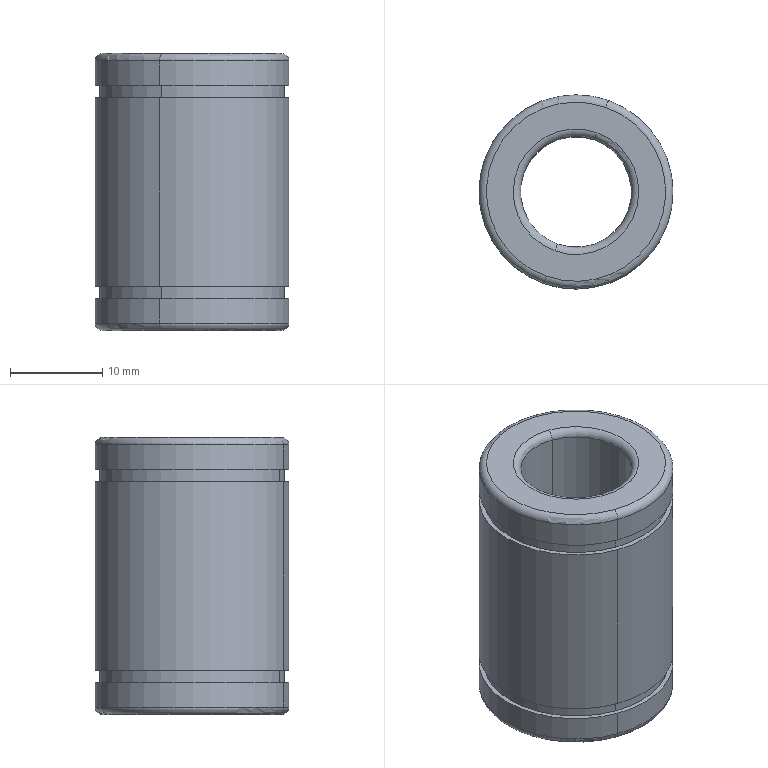Component | SolidWorks | LinearBearingLMUM12-3 | 1 solid | 26 faces | box 21 x 21 x 30 mm | volume 6886 mm3 | cylinder 12 | torus 8 | plane 6 | commonest cylinder face diameters 21 x6 20 x4 12 x2
build123d program:
from build123d import *

# Parameters (mm, degrees)
SKETCH1_R           = 10.5
SKETCH1_R_2         = 6
BOSS_EXTRUDE1_DEPTH = 30
SKETCH2_W           = 1.3
SKETCH2_H           = 0.5
FILLET2_R           = 0.8


with BuildPart() as part:
    # Sketch1 → Boss-Extrude1 (new body)
    with BuildSketch(Plane.XY):
        Circle(SKETCH1_R)
        Circle(SKETCH1_R_2, mode=Mode.SUBTRACT)
    extrude(amount=BOSS_EXTRUDE1_DEPTH)

    # Sketch2 → Cut-Revolve1 (revolve, cut)
    with BuildSketch(Plane(origin=(0, 0, 0), x_dir=(0, 0, -1), z_dir=(1, 0, 0)), mode=Mode.PRIVATE) as cut_revolve1_sk:
        with Locations((-4.15, -10.25)):
            Rectangle(SKETCH2_W, SKETCH2_H)
        with Locations((-25.85, -10.25)):
            Rectangle(SKETCH2_W, SKETCH2_H)
    revolve(cut_revolve1_sk.sketch.rotate(Axis((0, 0, 0), (0, 0, 1)), 270), axis=Axis((0, 0, 0), (0, 0, 1)), mode=Mode.SUBTRACT)

    # Fillet2
    fillet2_edges = [part.edges().sort_by_distance(p)[0] for p in [
        (-10.5, 0, 0),
        (-10.5, 0, 30),
        (-6, 0, 0),
        (-6, 0, 30),
    ]]
    fillet(fillet2_edges, radius=FILLET2_R)


solid = part.part

# Placed as in the assembly
solid = solid.moved(Location((-13.181, -42.432, -15.2), (0, 0, 0)))
STEP:
#1=COLOUR_RGB('',0.7922,0.8196,0.9333);
#2=FILL_AREA_STYLE_COLOUR('',#1);
#3=FILL_AREA_STYLE('',(#2));
#4=SURFACE_STYLE_FILL_AREA(#3);
#5=SURFACE_SIDE_STYLE('',(#4));
#6=SURFACE_STYLE_USAGE(.BOTH.,#5);
#7=PRESENTATION_STYLE_ASSIGNMENT((#6));
#8=CARTESIAN_POINT('',(-0.6462,-2.031,-0.5984));
#9=VERTEX_POINT('',#8);
#10=CARTESIAN_POINT('',(-0.3916,-1.31,-0.5984));
#11=VERTEX_POINT('',#10);
#12=CARTESIAN_POINT('',(-0.5189,-1.671,-0.5984));
#13=DIRECTION('',(0.,0.,-1.));
#14=DIRECTION('',(0.3333,0.9428,0.));
#15=AXIS2_PLACEMENT_3D('',#12,#13,#14);
#16=CIRCLE('',#15,0.3819);
#17=EDGE_CURVE('',#9,#11,#16,.T.);
#18=ORIENTED_EDGE('',*,*,#17,.F.);
#19=CARTESIAN_POINT('',(-0.6567,-2.06,-0.5669));
#20=VERTEX_POINT('',#19);
#21=CARTESIAN_POINT('',(-0.6462,-2.031,-0.5669));
#22=DIRECTION('',(-0.9428,0.3333,0.));
#23=DIRECTION('',(-0.3333,-0.9428,0.));
#24=AXIS2_PLACEMENT_3D('',#21,#22,#23);
#25=CIRCLE('',#24,0.0315);
#26=EDGE_CURVE('',#9,#20,#25,.T.);
#27=ORIENTED_EDGE('',*,*,#26,.T.);
#28=CARTESIAN_POINT('',(-0.3811,-1.281,-0.5669));
#29=VERTEX_POINT('',#28);
#30=CARTESIAN_POINT('',(-0.5189,-1.671,-0.5669));
#31=DIRECTION('',(0.,0.,1.));
#32=DIRECTION('',(0.3333,0.9428,0.));
#33=AXIS2_PLACEMENT_3D('',#30,#31,#32);
#34=CIRCLE('',#33,0.4134);
#35=EDGE_CURVE('',#29,#20,#34,.T.);
#36=ORIENTED_EDGE('',*,*,#35,.F.);
#37=CARTESIAN_POINT('',(-0.3916,-1.31,-0.5669));
#38=DIRECTION('',(0.9428,-0.3333,0.));
#39=DIRECTION('',(0.3333,0.9428,0.));
#40=AXIS2_PLACEMENT_3D('',#37,#38,#39);
#41=CIRCLE('',#40,0.0315);
#42=EDGE_CURVE('',#11,#29,#41,.T.);
#43=ORIENTED_EDGE('',*,*,#42,.F.);
#44=EDGE_LOOP('',(#18,#27,#36,#43));
#45=FACE_OUTER_BOUND('',#44,.T.);
#46=CARTESIAN_POINT('',(-0.5189,-1.671,-0.5669));
#47=DIRECTION('',(0.,0.,1.));
#48=DIRECTION('',(0.3333,0.9428,0.));
#49=AXIS2_PLACEMENT_3D('',#46,#47,#48);
#50=TOROIDAL_SURFACE('',#49,0.3819,0.0315);
#51=ADVANCED_FACE('',(#45),#50,.T.);
#52=CARTESIAN_POINT('',(-0.5977,-1.893,-0.5669));
#53=VERTEX_POINT('',#52);
#54=CARTESIAN_POINT('',(-0.4402,-1.448,-0.5669));
#55=VERTEX_POINT('',#54);
#56=CARTESIAN_POINT('',(-0.5189,-1.671,-0.5669));
#57=DIRECTION('',(0.,0.,-1.));
#58=DIRECTION('',(0.3333,0.9428,0.));
#59=AXIS2_PLACEMENT_3D('',#56,#57,#58);
#60=CIRCLE('',#59,0.2362);
#61=EDGE_CURVE('',#53,#55,#60,.T.);
#62=ORIENTED_EDGE('',*,*,#61,.F.);
#63=CARTESIAN_POINT('',(-0.6082,-1.923,-0.5984));
#64=VERTEX_POINT('',#63);
#65=CARTESIAN_POINT('',(-0.6082,-1.923,-0.5669));
#66=DIRECTION('',(-0.9428,0.3333,0.));
#67=DIRECTION('',(-0.3333,-0.9428,0.));
#68=AXIS2_PLACEMENT_3D('',#65,#66,#67);
#69=CIRCLE('',#68,0.0315);
#70=EDGE_CURVE('',#53,#64,#69,.T.);
#71=ORIENTED_EDGE('',*,*,#70,.T.);
#72=CARTESIAN_POINT('',(-0.4297,-1.418,-0.5984));
#73=VERTEX_POINT('',#72);
#74=CARTESIAN_POINT('',(-0.5189,-1.671,-0.5984));
#75=DIRECTION('',(0.,0.,1.));
#76=DIRECTION('',(0.3333,0.9428,0.));
#77=AXIS2_PLACEMENT_3D('',#74,#75,#76);
#78=CIRCLE('',#77,0.2677);
#79=EDGE_CURVE('',#73,#64,#78,.T.);
#80=ORIENTED_EDGE('',*,*,#79,.F.);
#81=CARTESIAN_POINT('',(-0.4297,-1.418,-0.5669));
#82=DIRECTION('',(0.9428,-0.3333,0.));
#83=DIRECTION('',(0.3333,0.9428,0.));
#84=AXIS2_PLACEMENT_3D('',#81,#82,#83);
#85=CIRCLE('',#84,0.0315);
#86=EDGE_CURVE('',#55,#73,#85,.T.);
#87=ORIENTED_EDGE('',*,*,#86,.F.);
#88=EDGE_LOOP('',(#62,#71,#80,#87));
#89=FACE_OUTER_BOUND('',#88,.T.);
#90=CARTESIAN_POINT('',(-0.5189,-1.671,-0.5669));
#91=DIRECTION('',(0.,0.,1.));
#92=DIRECTION('',(0.3333,0.9428,0.));
#93=AXIS2_PLACEMENT_3D('',#90,#91,#92);
#94=TOROIDAL_SURFACE('',#93,0.2677,0.0315);
#95=ADVANCED_FACE('',(#89),#94,.T.);
#96=CARTESIAN_POINT('',(-0.6567,-2.06,0.5512));
#97=VERTEX_POINT('',#96);
#98=CARTESIAN_POINT('',(-0.3811,-1.281,0.5512));
#99=VERTEX_POINT('',#98);
#100=CARTESIAN_POINT('',(-0.5189,-1.671,0.5512));
#101=DIRECTION('',(0.,0.,-1.));
#102=DIRECTION('',(0.3333,0.9428,0.));
#103=AXIS2_PLACEMENT_3D('',#100,#101,#102);
#104=CIRCLE('',#103,0.4134);
#105=EDGE_CURVE('',#97,#99,#104,.T.);
#106=ORIENTED_EDGE('',*,*,#105,.F.);
#107=CARTESIAN_POINT('',(-0.6462,-2.031,0.5827));
#108=VERTEX_POINT('',#107);
#109=CARTESIAN_POINT('',(-0.6462,-2.031,0.5512));
#110=DIRECTION('',(-0.9428,0.3333,0.));
#111=DIRECTION('',(-0.3333,-0.9428,0.));
#112=AXIS2_PLACEMENT_3D('',#109,#110,#111);
#113=CIRCLE('',#112,0.0315);
#114=EDGE_CURVE('',#97,#108,#113,.T.);
#115=ORIENTED_EDGE('',*,*,#114,.T.);
#116=CARTESIAN_POINT('',(-0.3916,-1.31,0.5827));
#117=VERTEX_POINT('',#116);
#118=CARTESIAN_POINT('',(-0.5189,-1.671,0.5827));
#119=DIRECTION('',(0.,0.,1.));
#120=DIRECTION('',(0.3333,0.9428,0.));
#121=AXIS2_PLACEMENT_3D('',#118,#119,#120);
#122=CIRCLE('',#121,0.3819);
#123=EDGE_CURVE('',#117,#108,#122,.T.);
#124=ORIENTED_EDGE('',*,*,#123,.F.);
#125=CARTESIAN_POINT('',(-0.3916,-1.31,0.5512));
#126=DIRECTION('',(0.9428,-0.3333,0.));
#127=DIRECTION('',(0.3333,0.9428,0.));
#128=AXIS2_PLACEMENT_3D('',#125,#126,#127);
#129=CIRCLE('',#128,0.0315);
#130=EDGE_CURVE('',#99,#117,#129,.T.);
#131=ORIENTED_EDGE('',*,*,#130,.F.);
#132=EDGE_LOOP('',(#106,#115,#124,#131));
#133=FACE_OUTER_BOUND('',#132,.T.);
#134=CARTESIAN_POINT('',(-0.5189,-1.671,0.5512));
#135=DIRECTION('',(0.,0.,1.));
#136=DIRECTION('',(0.3333,0.9428,0.));
#137=AXIS2_PLACEMENT_3D('',#134,#135,#136);
#138=TOROIDAL_SURFACE('',#137,0.3819,0.0315);
#139=ADVANCED_FACE('',(#133),#138,.T.);
#140=CARTESIAN_POINT('',(-0.6082,-1.923,0.5827));
#141=VERTEX_POINT('',#140);
#142=CARTESIAN_POINT('',(-0.4297,-1.418,0.5827));
#143=VERTEX_POINT('',#142);
#144=CARTESIAN_POINT('',(-0.5189,-1.671,0.5827));
#145=DIRECTION('',(0.,0.,-1.));
#146=DIRECTION('',(0.3333,0.9428,0.));
#147=AXIS2_PLACEMENT_3D('',#144,#145,#146);
#148=CIRCLE('',#147,0.2677);
#149=EDGE_CURVE('',#141,#143,#148,.T.);
#150=ORIENTED_EDGE('',*,*,#149,.F.);
#151=CARTESIAN_POINT('',(-0.5977,-1.893,0.5512));
#152=VERTEX_POINT('',#151);
#153=CARTESIAN_POINT('',(-0.6082,-1.923,0.5512));
#154=DIRECTION('',(-0.9428,0.3333,0.));
#155=DIRECTION('',(-0.3333,-0.9428,0.));
#156=AXIS2_PLACEMENT_3D('',#153,#154,#155);
#157=CIRCLE('',#156,0.0315);
#158=EDGE_CURVE('',#141,#152,#157,.T.);
#159=ORIENTED_EDGE('',*,*,#158,.T.);
#160=CARTESIAN_POINT('',(-0.4402,-1.448,0.5512));
#161=VERTEX_POINT('',#160);
#162=CARTESIAN_POINT('',(-0.5189,-1.671,0.5512));
#163=DIRECTION('',(0.,0.,1.));
#164=DIRECTION('',(0.3333,0.9428,0.));
#165=AXIS2_PLACEMENT_3D('',#162,#163,#164);
#166=CIRCLE('',#165,0.2362);
#167=EDGE_CURVE('',#161,#152,#166,.T.);
#168=ORIENTED_EDGE('',*,*,#167,.F.);
#169=CARTESIAN_POINT('',(-0.4297,-1.418,0.5512));
#170=DIRECTION('',(0.9428,-0.3333,0.));
#171=DIRECTION('',(0.3333,0.9428,0.));
#172=AXIS2_PLACEMENT_3D('',#169,#170,#171);
#173=CIRCLE('',#172,0.0315);
#174=EDGE_CURVE('',#143,#161,#173,.T.);
#175=ORIENTED_EDGE('',*,*,#174,.F.);
#176=EDGE_LOOP('',(#150,#159,#168,#175));
#177=FACE_OUTER_BOUND('',#176,.T.);
#178=CARTESIAN_POINT('',(-0.5189,-1.671,0.5512));
#179=DIRECTION('',(0.,0.,1.));
#180=DIRECTION('',(0.3333,0.9428,0.));
#181=AXIS2_PLACEMENT_3D('',#178,#179,#180);
#182=TOROIDAL_SURFACE('',#181,0.2677,0.0315);
#183=ADVANCED_FACE('',(#177),#182,.T.);
#184=CARTESIAN_POINT('',(-0.6501,-2.042,0.4449));
#185=VERTEX_POINT('',#184);
#186=CARTESIAN_POINT('',(-0.3877,-1.299,0.4449));
#187=VERTEX_POINT('',#186);
#188=CARTESIAN_POINT('',(-0.5189,-1.671,0.4449));
#189=DIRECTION('',(0.,0.,-1.));
#190=DIRECTION('',(-0.3333,-0.9428,0.));
#191=AXIS2_PLACEMENT_3D('',#188,#189,#190);
#192=CIRCLE('',#191,0.3937);
#193=EDGE_CURVE('',#185,#187,#192,.T.);
#194=ORIENTED_EDGE('',*,*,#193,.T.);
#195=CARTESIAN_POINT('',(-0.3877,-1.299,0.3937));
#196=VERTEX_POINT('',#195);
#197=CARTESIAN_POINT('',(-0.3877,-1.299,-0.5984));
#198=DIRECTION('',(0.,0.,-1.));
#199=VECTOR('',#198,39.37);
#200=LINE('',#197,#199);
#201=EDGE_CURVE('',#187,#196,#200,.T.);
#202=ORIENTED_EDGE('',*,*,#201,.T.);
#203=CARTESIAN_POINT('',(-0.6501,-2.042,0.3937));
#204=VERTEX_POINT('',#203);
#205=CARTESIAN_POINT('',(-0.5189,-1.671,0.3937));
#206=DIRECTION('',(0.,0.,-1.));
#207=DIRECTION('',(-0.3333,-0.9428,0.));
#208=AXIS2_PLACEMENT_3D('',#205,#206,#207);
#209=CIRCLE('',#208,0.3937);
#210=EDGE_CURVE('',#204,#196,#209,.T.);
#211=ORIENTED_EDGE('',*,*,#210,.F.);
#212=CARTESIAN_POINT('',(-0.6501,-2.042,-0.5984));
#213=DIRECTION('',(0.,0.,-1.));
#214=VECTOR('',#213,39.37);
#215=LINE('',#212,#214);
#216=EDGE_CURVE('',#185,#204,#215,.T.);
#217=ORIENTED_EDGE('',*,*,#216,.F.);
#218=EDGE_LOOP('',(#194,#202,#211,#217));
#219=FACE_OUTER_BOUND('',#218,.T.);
#220=CARTESIAN_POINT('',(-0.5189,-1.671,-0.5984));
#221=DIRECTION('',(0.,0.,-1.));
#222=DIRECTION('',(-0.3333,-0.9428,0.));
#223=AXIS2_PLACEMENT_3D('',#220,#221,#222);
#224=CYLINDRICAL_SURFACE('',#223,0.3937);
#225=ADVANCED_FACE('',(#219),#224,.T.);
#226=CARTESIAN_POINT('',(-0.6501,-2.042,-0.4094));
#227=VERTEX_POINT('',#226);
#228=CARTESIAN_POINT('',(-0.3877,-1.299,-0.4094));
#229=VERTEX_POINT('',#228);
#230=CARTESIAN_POINT('',(-0.5189,-1.671,-0.4094));
#231=DIRECTION('',(0.,0.,-1.));
#232=DIRECTION('',(-0.3333,-0.9428,0.));
#233=AXIS2_PLACEMENT_3D('',#230,#231,#232);
#234=CIRCLE('',#233,0.3937);
#235=EDGE_CURVE('',#227,#229,#234,.T.);
#236=ORIENTED_EDGE('',*,*,#235,.T.);
#237=CARTESIAN_POINT('',(-0.3877,-1.299,-0.4606));
#238=VERTEX_POINT('',#237);
#239=CARTESIAN_POINT('',(-0.3877,-1.299,-0.5984));
#240=DIRECTION('',(0.,0.,-1.));
#241=VECTOR('',#240,39.37);
#242=LINE('',#239,#241);
#243=EDGE_CURVE('',#229,#238,#242,.T.);
#244=ORIENTED_EDGE('',*,*,#243,.T.);
#245=CARTESIAN_POINT('',(-0.6501,-2.042,-0.4606));
#246=VERTEX_POINT('',#245);
#247=CARTESIAN_POINT('',(-0.5189,-1.671,-0.4606));
#248=DIRECTION('',(0.,0.,-1.));
#249=DIRECTION('',(-0.3333,-0.9428,0.));
#250=AXIS2_PLACEMENT_3D('',#247,#248,#249);
#251=CIRCLE('',#250,0.3937);
#252=EDGE_CURVE('',#246,#238,#251,.T.);
#253=ORIENTED_EDGE('',*,*,#252,.F.);
#254=CARTESIAN_POINT('',(-0.6501,-2.042,-0.5984));
#255=DIRECTION('',(0.,0.,-1.));
#256=VECTOR('',#255,39.37);
#257=LINE('',#254,#256);
#258=EDGE_CURVE('',#227,#246,#257,.T.);
#259=ORIENTED_EDGE('',*,*,#258,.F.);
#260=EDGE_LOOP('',(#236,#244,#253,#259));
#261=FACE_OUTER_BOUND('',#260,.T.);
#262=CARTESIAN_POINT('',(-0.5189,-1.671,-0.5984));
#263=DIRECTION('',(0.,0.,-1.));
#264=DIRECTION('',(-0.3333,-0.9428,0.));
#265=AXIS2_PLACEMENT_3D('',#262,#263,#264);
#266=CYLINDRICAL_SURFACE('',#265,0.3937);
#267=ADVANCED_FACE('',(#261),#266,.T.);
#268=CARTESIAN_POINT('',(-0.5189,-1.671,0.5512));
#269=DIRECTION('',(0.,0.,1.));
#270=DIRECTION('',(0.3333,0.9428,0.));
#271=AXIS2_PLACEMENT_3D('',#268,#269,#270);
#272=CIRCLE('',#271,0.2362);
#273=EDGE_CURVE('',#152,#161,#272,.T.);
#274=ORIENTED_EDGE('',*,*,#273,.T.);
#275=CARTESIAN_POINT('',(-0.4402,-1.448,0.5827));
#276=DIRECTION('',(0.,0.,-1.));
#277=VECTOR('',#276,39.37);
#278=LINE('',#275,#277);
#279=EDGE_CURVE('',#161,#55,#278,.T.);
#280=ORIENTED_EDGE('',*,*,#279,.T.);
#281=CARTESIAN_POINT('',(-0.5189,-1.671,-0.5669));
#282=DIRECTION('',(0.,0.,-1.));
#283=DIRECTION('',(0.3333,0.9428,0.));
#284=AXIS2_PLACEMENT_3D('',#281,#282,#283);
#285=CIRCLE('',#284,0.2362);
#286=EDGE_CURVE('',#55,#53,#285,.T.);
#287=ORIENTED_EDGE('',*,*,#286,.T.);
#288=CARTESIAN_POINT('',(-0.5977,-1.893,0.5827));
#289=DIRECTION('',(0.,0.,-1.));
#290=VECTOR('',#289,39.37);
#291=LINE('',#288,#290);
#292=EDGE_CURVE('',#152,#53,#291,.T.);
#293=ORIENTED_EDGE('',*,*,#292,.F.);
#294=EDGE_LOOP('',(#274,#280,#287,#293));
#295=FACE_OUTER_BOUND('',#294,.T.);
#296=CARTESIAN_POINT('',(-0.5189,-1.671,0.5827));
#297=DIRECTION('',(0.,0.,-1.));
#298=DIRECTION('',(-0.3333,-0.9428,0.));
#299=AXIS2_PLACEMENT_3D('',#296,#297,#298);
#300=CYLINDRICAL_SURFACE('',#299,0.2362);
#301=ADVANCED_FACE('',(#295),#300,.F.);
#302=CARTESIAN_POINT('',(-0.6567,-2.06,-0.4606));
#303=VERTEX_POINT('',#302);
#304=CARTESIAN_POINT('',(-0.3811,-1.281,-0.4606));
#305=VERTEX_POINT('',#304);
#306=CARTESIAN_POINT('',(-0.5189,-1.671,-0.4606));
#307=DIRECTION('',(0.,0.,-1.));
#308=DIRECTION('',(-0.3333,-0.9428,0.));
#309=AXIS2_PLACEMENT_3D('',#306,#307,#308);
#310=CIRCLE('',#309,0.4134);
#311=EDGE_CURVE('',#303,#305,#310,.T.);
#312=ORIENTED_EDGE('',*,*,#311,.T.);
#313=CARTESIAN_POINT('',(-0.3811,-1.281,0.5827));
#314=DIRECTION('',(0.,0.,-1.));
#315=VECTOR('',#314,39.37);
#316=LINE('',#313,#315);
#317=EDGE_CURVE('',#305,#29,#316,.T.);
#318=ORIENTED_EDGE('',*,*,#317,.T.);
#319=ORIENTED_EDGE('',*,*,#35,.T.);
#320=CARTESIAN_POINT('',(-0.6567,-2.06,0.5827));
#321=DIRECTION('',(0.,0.,-1.));
#322=VECTOR('',#321,39.37);
#323=LINE('',#320,#322);
#324=EDGE_CURVE('',#303,#20,#323,.T.);
#325=ORIENTED_EDGE('',*,*,#324,.F.);
#326=EDGE_LOOP('',(#312,#318,#319,#325));
#327=FACE_OUTER_BOUND('',#326,.T.);
#328=CARTESIAN_POINT('',(-0.5189,-1.671,0.5827));
#329=DIRECTION('',(0.,0.,-1.));
#330=DIRECTION('',(-0.3333,-0.9428,0.));
#331=AXIS2_PLACEMENT_3D('',#328,#329,#330);
#332=CYLINDRICAL_SURFACE('',#331,0.4134);
#333=ADVANCED_FACE('',(#327),#332,.T.);
#334=CARTESIAN_POINT('',(-0.6567,-2.06,0.3937));
#335=VERTEX_POINT('',#334);
#336=CARTESIAN_POINT('',(-0.3811,-1.281,0.3937));
#337=VERTEX_POINT('',#336);
#338=CARTESIAN_POINT('',(-0.5189,-1.671,0.3937));
#339=DIRECTION('',(0.,0.,-1.));
#340=DIRECTION('',(-0.3333,-0.9428,0.));
#341=AXIS2_PLACEMENT_3D('',#338,#339,#340);
#342=CIRCLE('',#341,0.4134);
#343=EDGE_CURVE('',#335,#337,#342,.T.);
#344=ORIENTED_EDGE('',*,*,#343,.T.);
#345=CARTESIAN_POINT('',(-0.3811,-1.281,-0.4094));
#346=VERTEX_POINT('',#345);
#347=CARTESIAN_POINT('',(-0.3811,-1.281,0.5827));
#348=DIRECTION('',(0.,0.,-1.));
#349=VECTOR('',#348,39.37);
#350=LINE('',#347,#349);
#351=EDGE_CURVE('',#337,#346,#350,.T.);
#352=ORIENTED_EDGE('',*,*,#351,.T.);
#353=CARTESIAN_POINT('',(-0.6567,-2.06,-0.4094));
#354=VERTEX_POINT('',#353);
#355=CARTESIAN_POINT('',(-0.5189,-1.671,-0.4094));
#356=DIRECTION('',(0.,0.,-1.));
#357=DIRECTION('',(-0.3333,-0.9428,0.));
#358=AXIS2_PLACEMENT_3D('',#355,#356,#357);
#359=CIRCLE('',#358,0.4134);
#360=EDGE_CURVE('',#354,#346,#359,.T.);
#361=ORIENTED_EDGE('',*,*,#360,.F.);
#362=CARTESIAN_POINT('',(-0.6567,-2.06,0.5827));
#363=DIRECTION('',(0.,0.,-1.));
#364=VECTOR('',#363,39.37);
#365=LINE('',#362,#364);
#366=EDGE_CURVE('',#335,#354,#365,.T.);
#367=ORIENTED_EDGE('',*,*,#366,.F.);
#368=EDGE_LOOP('',(#344,#352,#361,#367));
#369=FACE_OUTER_BOUND('',#368,.T.);
#370=CARTESIAN_POINT('',(-0.5189,-1.671,0.5827));
#371=DIRECTION('',(0.,0.,-1.));
#372=DIRECTION('',(-0.3333,-0.9428,0.));
#373=AXIS2_PLACEMENT_3D('',#370,#371,#372);
#374=CYLINDRICAL_SURFACE('',#373,0.4134);
#375=ADVANCED_FACE('',(#369),#374,.T.);
#376=ORIENTED_EDGE('',*,*,#105,.T.);
#377=CARTESIAN_POINT('',(-0.3811,-1.281,0.4449));
#378=VERTEX_POINT('',#377);
#379=CARTESIAN_POINT('',(-0.3811,-1.281,0.5827));
#380=DIRECTION('',(0.,0.,-1.));
#381=VECTOR('',#380,39.37);
#382=LINE('',#379,#381);
#383=EDGE_CURVE('',#99,#378,#382,.T.);
#384=ORIENTED_EDGE('',*,*,#383,.T.);
#385=CARTESIAN_POINT('',(-0.6567,-2.06,0.4449));
#386=VERTEX_POINT('',#385);
#387=CARTESIAN_POINT('',(-0.5189,-1.671,0.4449));
#388=DIRECTION('',(0.,0.,-1.));
#389=DIRECTION('',(-0.3333,-0.9428,0.));
#390=AXIS2_PLACEMENT_3D('',#387,#388,#389);
#391=CIRCLE('',#390,0.4134);
#392=EDGE_CURVE('',#386,#378,#391,.T.);
#393=ORIENTED_EDGE('',*,*,#392,.F.);
#394=CARTESIAN_POINT('',(-0.6567,-2.06,0.5827));
#395=DIRECTION('',(0.,0.,-1.));
#396=VECTOR('',#395,39.37);
#397=LINE('',#394,#396);
#398=EDGE_CURVE('',#97,#386,#397,.T.);
#399=ORIENTED_EDGE('',*,*,#398,.F.);
#400=EDGE_LOOP('',(#376,#384,#393,#399));
#401=FACE_OUTER_BOUND('',#400,.T.);
#402=CARTESIAN_POINT('',(-0.5189,-1.671,0.5827));
#403=DIRECTION('',(0.,0.,-1.));
#404=DIRECTION('',(-0.3333,-0.9428,0.));
#405=AXIS2_PLACEMENT_3D('',#402,#403,#404);
#406=CYLINDRICAL_SURFACE('',#405,0.4134);
#407=ADVANCED_FACE('',(#401),#406,.T.);
#408=ORIENTED_EDGE('',*,*,#383,.F.);
#409=CARTESIAN_POINT('',(-0.5189,-1.671,0.5512));
#410=DIRECTION('',(0.,0.,-1.));
#411=DIRECTION('',(0.3333,0.9428,0.));
#412=AXIS2_PLACEMENT_3D('',#409,#410,#411);
#413=CIRCLE('',#412,0.4134);
#414=EDGE_CURVE('',#99,#97,#413,.T.);
#415=ORIENTED_EDGE('',*,*,#414,.T.);
#416=ORIENTED_EDGE('',*,*,#398,.T.);
#417=CARTESIAN_POINT('',(-0.5189,-1.671,0.4449));
#418=DIRECTION('',(0.,0.,-1.));
#419=DIRECTION('',(-0.3333,-0.9428,0.));
#420=AXIS2_PLACEMENT_3D('',#417,#418,#419);
#421=CIRCLE('',#420,0.4134);
#422=EDGE_CURVE('',#378,#386,#421,.T.);
#423=ORIENTED_EDGE('',*,*,#422,.F.);
#424=EDGE_LOOP('',(#408,#415,#416,#423));
#425=FACE_OUTER_BOUND('',#424,.T.);
#426=CARTESIAN_POINT('',(-0.5189,-1.671,0.5827));
#427=DIRECTION('',(0.,0.,-1.));
#428=DIRECTION('',(-0.3333,-0.9428,0.));
#429=AXIS2_PLACEMENT_3D('',#426,#427,#428);
#430=CYLINDRICAL_SURFACE('',#429,0.4134);
#431=ADVANCED_FACE('',(#425),#430,.T.);
#432=ORIENTED_EDGE('',*,*,#351,.F.);
#433=CARTESIAN_POINT('',(-0.5189,-1.671,0.3937));
#434=DIRECTION('',(0.,0.,-1.));
#435=DIRECTION('',(-0.3333,-0.9428,0.));
#436=AXIS2_PLACEMENT_3D('',#433,#434,#435);
#437=CIRCLE('',#436,0.4134);
#438=EDGE_CURVE('',#337,#335,#437,.T.);
#439=ORIENTED_EDGE('',*,*,#438,.T.);
#440=ORIENTED_EDGE('',*,*,#366,.T.);
#441=CARTESIAN_POINT('',(-0.5189,-1.671,-0.4094));
#442=DIRECTION('',(0.,0.,-1.));
#443=DIRECTION('',(-0.3333,-0.9428,0.));
#444=AXIS2_PLACEMENT_3D('',#441,#442,#443);
#445=CIRCLE('',#444,0.4134);
#446=EDGE_CURVE('',#346,#354,#445,.T.);
#447=ORIENTED_EDGE('',*,*,#446,.F.);
#448=EDGE_LOOP('',(#432,#439,#440,#447));
#449=FACE_OUTER_BOUND('',#448,.T.);
#450=CARTESIAN_POINT('',(-0.5189,-1.671,0.5827));
#451=DIRECTION('',(0.,0.,-1.));
#452=DIRECTION('',(-0.3333,-0.9428,0.));
#453=AXIS2_PLACEMENT_3D('',#450,#451,#452);
#454=CYLINDRICAL_SURFACE('',#453,0.4134);
#455=ADVANCED_FACE('',(#449),#454,.T.);
#456=ORIENTED_EDGE('',*,*,#317,.F.);
#457=CARTESIAN_POINT('',(-0.5189,-1.671,-0.4606));
#458=DIRECTION('',(0.,0.,-1.));
#459=DIRECTION('',(-0.3333,-0.9428,0.));
#460=AXIS2_PLACEMENT_3D('',#457,#458,#459);
#461=CIRCLE('',#460,0.4134);
#462=EDGE_CURVE('',#305,#303,#461,.T.);
#463=ORIENTED_EDGE('',*,*,#462,.T.);
#464=ORIENTED_EDGE('',*,*,#324,.T.);
#465=CARTESIAN_POINT('',(-0.5189,-1.671,-0.5669));
#466=DIRECTION('',(0.,0.,1.));
#467=DIRECTION('',(0.3333,0.9428,0.));
#468=AXIS2_PLACEMENT_3D('',#465,#466,#467);
#469=CIRCLE('',#468,0.4134);
#470=EDGE_CURVE('',#20,#29,#469,.T.);
#471=ORIENTED_EDGE('',*,*,#470,.T.);
#472=EDGE_LOOP('',(#456,#463,#464,#471));
#473=FACE_OUTER_BOUND('',#472,.T.);
#474=CARTESIAN_POINT('',(-0.5189,-1.671,0.5827));
#475=DIRECTION('',(0.,0.,-1.));
#476=DIRECTION('',(-0.3333,-0.9428,0.));
#477=AXIS2_PLACEMENT_3D('',#474,#475,#476);
#478=CYLINDRICAL_SURFACE('',#477,0.4134);
#479=ADVANCED_FACE('',(#473),#478,.T.);
#480=CARTESIAN_POINT('',(-0.5189,-1.671,0.5827));
#481=DIRECTION('',(0.,0.,-1.));
#482=DIRECTION('',(0.3333,0.9428,0.));
#483=AXIS2_PLACEMENT_3D('',#480,#481,#482);
#484=CIRCLE('',#483,0.2677);
#485=EDGE_CURVE('',#143,#141,#484,.T.);
#486=ORIENTED_EDGE('',*,*,#485,.T.);
#487=ORIENTED_EDGE('',*,*,#149,.T.);
#488=EDGE_LOOP('',(#486,#487));
#489=FACE_BOUND('',#488,.T.);
#490=ORIENTED_EDGE('',*,*,#123,.T.);
#491=CARTESIAN_POINT('',(-0.5189,-1.671,0.5827));
#492=DIRECTION('',(0.,0.,1.));
#493=DIRECTION('',(0.3333,0.9428,0.));
#494=AXIS2_PLACEMENT_3D('',#491,#492,#493);
#495=CIRCLE('',#494,0.3819);
#496=EDGE_CURVE('',#108,#117,#495,.T.);
#497=ORIENTED_EDGE('',*,*,#496,.T.);
#498=EDGE_LOOP('',(#490,#497));
#499=FACE_OUTER_BOUND('',#498,.T.);
#500=CARTESIAN_POINT('',(-0.5189,-1.671,0.5827));
#501=DIRECTION('',(0.,0.,1.));
#502=DIRECTION('',(0.3333,0.9428,0.));
#503=AXIS2_PLACEMENT_3D('',#500,#501,#502);
#504=PLANE('',#503);
#505=ADVANCED_FACE('',(#489,#499),#504,.T.);
#506=ORIENTED_EDGE('',*,*,#79,.T.);
#507=CARTESIAN_POINT('',(-0.5189,-1.671,-0.5984));
#508=DIRECTION('',(0.,0.,1.));
#509=DIRECTION('',(0.3333,0.9428,0.));
#510=AXIS2_PLACEMENT_3D('',#507,#508,#509);
#511=CIRCLE('',#510,0.2677);
#512=EDGE_CURVE('',#64,#73,#511,.T.);
#513=ORIENTED_EDGE('',*,*,#512,.T.);
#514=EDGE_LOOP('',(#506,#513));
#515=FACE_BOUND('',#514,.T.);
#516=CARTESIAN_POINT('',(-0.5189,-1.671,-0.5984));
#517=DIRECTION('',(0.,0.,-1.));
#518=DIRECTION('',(0.3333,0.9428,0.));
#519=AXIS2_PLACEMENT_3D('',#516,#517,#518);
#520=CIRCLE('',#519,0.3819);
#521=EDGE_CURVE('',#11,#9,#520,.T.);
#522=ORIENTED_EDGE('',*,*,#521,.T.);
#523=ORIENTED_EDGE('',*,*,#17,.T.);
#524=EDGE_LOOP('',(#522,#523));
#525=FACE_OUTER_BOUND('',#524,.T.);
#526=CARTESIAN_POINT('',(-0.5189,-1.671,-0.5984));
#527=DIRECTION('',(0.,0.,1.));
#528=DIRECTION('',(0.3333,0.9428,0.));
#529=AXIS2_PLACEMENT_3D('',#526,#527,#528);
#530=PLANE('',#529);
#531=ADVANCED_FACE('',(#515,#525),#530,.F.);
#532=ORIENTED_EDGE('',*,*,#279,.F.);
#533=ORIENTED_EDGE('',*,*,#167,.T.);
#534=ORIENTED_EDGE('',*,*,#292,.T.);
#535=ORIENTED_EDGE('',*,*,#61,.T.);
#536=EDGE_LOOP('',(#532,#533,#534,#535));
#537=FACE_OUTER_BOUND('',#536,.T.);
#538=CARTESIAN_POINT('',(-0.5189,-1.671,0.5827));
#539=DIRECTION('',(0.,0.,-1.));
#540=DIRECTION('',(-0.3333,-0.9428,0.));
#541=AXIS2_PLACEMENT_3D('',#538,#539,#540);
#542=CYLINDRICAL_SURFACE('',#541,0.2362);
#543=ADVANCED_FACE('',(#537),#542,.F.);
#544=ORIENTED_EDGE('',*,*,#360,.T.);
#545=ORIENTED_EDGE('',*,*,#446,.T.);
#546=EDGE_LOOP('',(#544,#545));
#547=FACE_OUTER_BOUND('',#546,.T.);
#548=ORIENTED_EDGE('',*,*,#235,.F.);
#549=CARTESIAN_POINT('',(-0.5189,-1.671,-0.4094));
#550=DIRECTION('',(0.,0.,-1.));
#551=DIRECTION('',(-0.3333,-0.9428,0.));
#552=AXIS2_PLACEMENT_3D('',#549,#550,#551);
#553=CIRCLE('',#552,0.3937);
#554=EDGE_CURVE('',#229,#227,#553,.T.);
#555=ORIENTED_EDGE('',*,*,#554,.F.);
#556=EDGE_LOOP('',(#548,#555));
#557=FACE_BOUND('',#556,.T.);
#558=CARTESIAN_POINT('',(-0.1292,-1.808,-0.4094));
#559=DIRECTION('',(0.,0.,-1.));
#560=DIRECTION('',(-0.3333,-0.9428,0.));
#561=AXIS2_PLACEMENT_3D('',#558,#559,#560);
#562=PLANE('',#561);
#563=ADVANCED_FACE('',(#547,#557),#562,.T.);
#564=ORIENTED_EDGE('',*,*,#243,.F.);
#565=ORIENTED_EDGE('',*,*,#554,.T.);
#566=ORIENTED_EDGE('',*,*,#258,.T.);
#567=CARTESIAN_POINT('',(-0.5189,-1.671,-0.4606));
#568=DIRECTION('',(0.,0.,-1.));
#569=DIRECTION('',(-0.3333,-0.9428,0.));
#570=AXIS2_PLACEMENT_3D('',#567,#568,#569);
#571=CIRCLE('',#570,0.3937);
#572=EDGE_CURVE('',#238,#246,#571,.T.);
#573=ORIENTED_EDGE('',*,*,#572,.F.);
#574=EDGE_LOOP('',(#564,#565,#566,#573));
#575=FACE_OUTER_BOUND('',#574,.T.);
#576=CARTESIAN_POINT('',(-0.5189,-1.671,-0.5984));
#577=DIRECTION('',(0.,0.,-1.));
#578=DIRECTION('',(-0.3333,-0.9428,0.));
#579=AXIS2_PLACEMENT_3D('',#576,#577,#578);
#580=CYLINDRICAL_SURFACE('',#579,0.3937);
#581=ADVANCED_FACE('',(#575),#580,.T.);
#582=ORIENTED_EDGE('',*,*,#252,.T.);
#583=ORIENTED_EDGE('',*,*,#572,.T.);
#584=EDGE_LOOP('',(#582,#583));
#585=FACE_BOUND('',#584,.T.);
#586=ORIENTED_EDGE('',*,*,#311,.F.);
#587=ORIENTED_EDGE('',*,*,#462,.F.);
#588=EDGE_LOOP('',(#586,#587));
#589=FACE_OUTER_BOUND('',#588,.T.);
#590=CARTESIAN_POINT('',(-0.1292,-1.808,-0.4606));
#591=DIRECTION('',(0.,0.,1.));
#592=DIRECTION('',(0.3333,0.9428,0.));
#593=AXIS2_PLACEMENT_3D('',#590,#591,#592);
#594=PLANE('',#593);
#595=ADVANCED_FACE('',(#585,#589),#594,.T.);
#596=ORIENTED_EDGE('',*,*,#392,.T.);
#597=ORIENTED_EDGE('',*,*,#422,.T.);
#598=EDGE_LOOP('',(#596,#597));
#599=FACE_OUTER_BOUND('',#598,.T.);
#600=ORIENTED_EDGE('',*,*,#193,.F.);
#601=CARTESIAN_POINT('',(-0.5189,-1.671,0.4449));
#602=DIRECTION('',(0.,0.,-1.));
#603=DIRECTION('',(-0.3333,-0.9428,0.));
#604=AXIS2_PLACEMENT_3D('',#601,#602,#603);
#605=CIRCLE('',#604,0.3937);
#606=EDGE_CURVE('',#187,#185,#605,.T.);
#607=ORIENTED_EDGE('',*,*,#606,.F.);
#608=EDGE_LOOP('',(#600,#607));
#609=FACE_BOUND('',#608,.T.);
#610=CARTESIAN_POINT('',(-0.1292,-1.808,0.4449));
#611=DIRECTION('',(0.,0.,-1.));
#612=DIRECTION('',(-0.3333,-0.9428,0.));
#613=AXIS2_PLACEMENT_3D('',#610,#611,#612);
#614=PLANE('',#613);
#615=ADVANCED_FACE('',(#599,#609),#614,.T.);
#616=ORIENTED_EDGE('',*,*,#201,.F.);
#617=ORIENTED_EDGE('',*,*,#606,.T.);
#618=ORIENTED_EDGE('',*,*,#216,.T.);
#619=CARTESIAN_POINT('',(-0.5189,-1.671,0.3937));
#620=DIRECTION('',(0.,0.,-1.));
#621=DIRECTION('',(-0.3333,-0.9428,0.));
#622=AXIS2_PLACEMENT_3D('',#619,#620,#621);
#623=CIRCLE('',#622,0.3937);
#624=EDGE_CURVE('',#196,#204,#623,.T.);
#625=ORIENTED_EDGE('',*,*,#624,.F.);
#626=EDGE_LOOP('',(#616,#617,#618,#625));
#627=FACE_OUTER_BOUND('',#626,.T.);
#628=CARTESIAN_POINT('',(-0.5189,-1.671,-0.5984));
#629=DIRECTION('',(0.,0.,-1.));
#630=DIRECTION('',(-0.3333,-0.9428,0.));
#631=AXIS2_PLACEMENT_3D('',#628,#629,#630);
#632=CYLINDRICAL_SURFACE('',#631,0.3937);
#633=ADVANCED_FACE('',(#627),#632,.T.);
#634=ORIENTED_EDGE('',*,*,#210,.T.);
#635=ORIENTED_EDGE('',*,*,#624,.T.);
#636=EDGE_LOOP('',(#634,#635));
#637=FACE_BOUND('',#636,.T.);
#638=ORIENTED_EDGE('',*,*,#343,.F.);
#639=ORIENTED_EDGE('',*,*,#438,.F.);
#640=EDGE_LOOP('',(#638,#639));
#641=FACE_OUTER_BOUND('',#640,.T.);
#642=CARTESIAN_POINT('',(-0.1292,-1.808,0.3937));
#643=DIRECTION('',(0.,0.,1.));
#644=DIRECTION('',(0.3333,0.9428,0.));
#645=AXIS2_PLACEMENT_3D('',#642,#643,#644);
#646=PLANE('',#645);
#647=ADVANCED_FACE('',(#637,#641),#646,.T.);
#648=ORIENTED_EDGE('',*,*,#158,.F.);
#649=ORIENTED_EDGE('',*,*,#485,.F.);
#650=ORIENTED_EDGE('',*,*,#174,.T.);
#651=ORIENTED_EDGE('',*,*,#273,.F.);
#652=EDGE_LOOP('',(#648,#649,#650,#651));
#653=FACE_OUTER_BOUND('',#652,.T.);
#654=CARTESIAN_POINT('',(-0.5189,-1.671,0.5512));
#655=DIRECTION('',(0.,0.,1.));
#656=DIRECTION('',(0.3333,0.9428,0.));
#657=AXIS2_PLACEMENT_3D('',#654,#655,#656);
#658=TOROIDAL_SURFACE('',#657,0.2677,0.0315);
#659=ADVANCED_FACE('',(#653),#658,.T.);
#660=ORIENTED_EDGE('',*,*,#114,.F.);
#661=ORIENTED_EDGE('',*,*,#414,.F.);
#662=ORIENTED_EDGE('',*,*,#130,.T.);
#663=ORIENTED_EDGE('',*,*,#496,.F.);
#664=EDGE_LOOP('',(#660,#661,#662,#663));
#665=FACE_OUTER_BOUND('',#664,.T.);
#666=CARTESIAN_POINT('',(-0.5189,-1.671,0.5512));
#667=DIRECTION('',(0.,0.,1.));
#668=DIRECTION('',(0.3333,0.9428,0.));
#669=AXIS2_PLACEMENT_3D('',#666,#667,#668);
#670=TOROIDAL_SURFACE('',#669,0.3819,0.0315);
#671=ADVANCED_FACE('',(#665),#670,.T.);
#672=ORIENTED_EDGE('',*,*,#70,.F.);
#673=ORIENTED_EDGE('',*,*,#286,.F.);
#674=ORIENTED_EDGE('',*,*,#86,.T.);
#675=ORIENTED_EDGE('',*,*,#512,.F.);
#676=EDGE_LOOP('',(#672,#673,#674,#675));
#677=FACE_OUTER_BOUND('',#676,.T.);
#678=CARTESIAN_POINT('',(-0.5189,-1.671,-0.5669));
#679=DIRECTION('',(0.,0.,1.));
#680=DIRECTION('',(0.3333,0.9428,0.));
#681=AXIS2_PLACEMENT_3D('',#678,#679,#680);
#682=TOROIDAL_SURFACE('',#681,0.2677,0.0315);
#683=ADVANCED_FACE('',(#677),#682,.T.);
#684=ORIENTED_EDGE('',*,*,#26,.F.);
#685=ORIENTED_EDGE('',*,*,#521,.F.);
#686=ORIENTED_EDGE('',*,*,#42,.T.);
#687=ORIENTED_EDGE('',*,*,#470,.F.);
#688=EDGE_LOOP('',(#684,#685,#686,#687));
#689=FACE_OUTER_BOUND('',#688,.T.);
#690=CARTESIAN_POINT('',(-0.5189,-1.671,-0.5669));
#691=DIRECTION('',(0.,0.,1.));
#692=DIRECTION('',(0.3333,0.9428,0.));
#693=AXIS2_PLACEMENT_3D('',#690,#691,#692);
#694=TOROIDAL_SURFACE('',#693,0.3819,0.0315);
#695=ADVANCED_FACE('',(#689),#694,.T.);
#696=CLOSED_SHELL('',(#51,#95,#139,#183,#225,#267,#301,#333,#375,#407,#431,#455,#479,#505,#531,#543,#563,#581,#595,#615,#633,#647,#659,#671,#683,#695));
#697=MANIFOLD_SOLID_BREP('',#696);
#698=STYLED_ITEM('',(#7),#697);
#699=(LENGTH_UNIT()NAMED_UNIT(*)SI_UNIT($,.METRE.));
#700=LENGTH_MEASURE_WITH_UNIT(LENGTH_MEASURE(0.0254),#699);
#701=DIMENSIONAL_EXPONENTS(1.,0.,0.,0.,0.,0.,0.);
#702=(CONVERSION_BASED_UNIT('',#700)LENGTH_UNIT()NAMED_UNIT(#701));
#703=UNCERTAINTY_MEASURE_WITH_UNIT(LENGTH_MEASURE(0.00001),#702,'','');
#704=(NAMED_UNIT(*)PLANE_ANGLE_UNIT()SI_UNIT($,.RADIAN.));
#705=(NAMED_UNIT(*)SI_UNIT($,.STERADIAN.)SOLID_ANGLE_UNIT());
#706=(GEOMETRIC_REPRESENTATION_CONTEXT(3)GLOBAL_UNCERTAINTY_ASSIGNED_CONTEXT((#703))GLOBAL_UNIT_ASSIGNED_CONTEXT((#702,#704,#705))REPRESENTATION_CONTEXT('',''));
#707=MECHANICAL_DESIGN_GEOMETRIC_PRESENTATION_REPRESENTATION('',(#698),#706);
#708=PRESENTATION_LAYER_ASSIGNMENT('','',(#698));
#709=CARTESIAN_POINT('',(0.,0.,0.));
#710=DIRECTION('',(0.,0.,1.));
#711=DIRECTION('',(1.,0.,0.));
#712=AXIS2_PLACEMENT_3D('',#709,#710,#711);
#713=(LENGTH_UNIT()NAMED_UNIT(*)SI_UNIT($,.METRE.));
#714=LENGTH_MEASURE_WITH_UNIT(LENGTH_MEASURE(0.0254),#713);
#715=DIMENSIONAL_EXPONENTS(1.,0.,0.,0.,0.,0.,0.);
#716=(CONVERSION_BASED_UNIT('',#714)LENGTH_UNIT()NAMED_UNIT(#715));
#717=UNCERTAINTY_MEASURE_WITH_UNIT(LENGTH_MEASURE(0.00001),#716,'','');
#718=(NAMED_UNIT(*)PLANE_ANGLE_UNIT()SI_UNIT($,.RADIAN.));
#719=(NAMED_UNIT(*)SI_UNIT($,.STERADIAN.)SOLID_ANGLE_UNIT());
#720=(GEOMETRIC_REPRESENTATION_CONTEXT(3)GLOBAL_UNCERTAINTY_ASSIGNED_CONTEXT((#717))GLOBAL_UNIT_ASSIGNED_CONTEXT((#716,#718,#719))REPRESENTATION_CONTEXT('',''));
#721=ADVANCED_BREP_SHAPE_REPRESENTATION('',(#697,#712),#720);